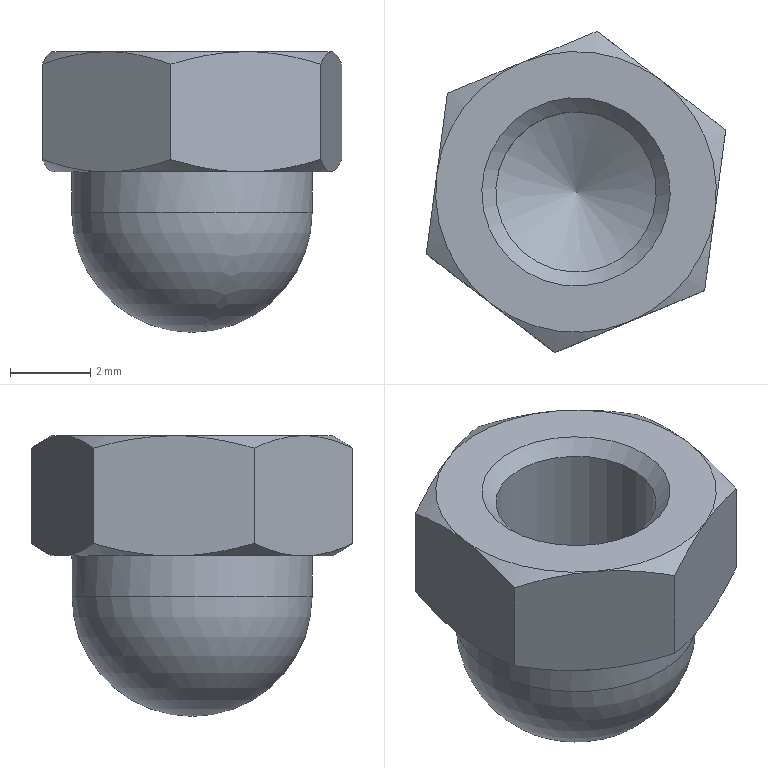Component | NX | FLANGE_NUT_M4 | 1 solid | 25 faces | volume 149 mm3 | cone 14 | plane 8 | cylinder 2 | sphere 1 | commonest cylinder face diameters 4 x1 6 x1